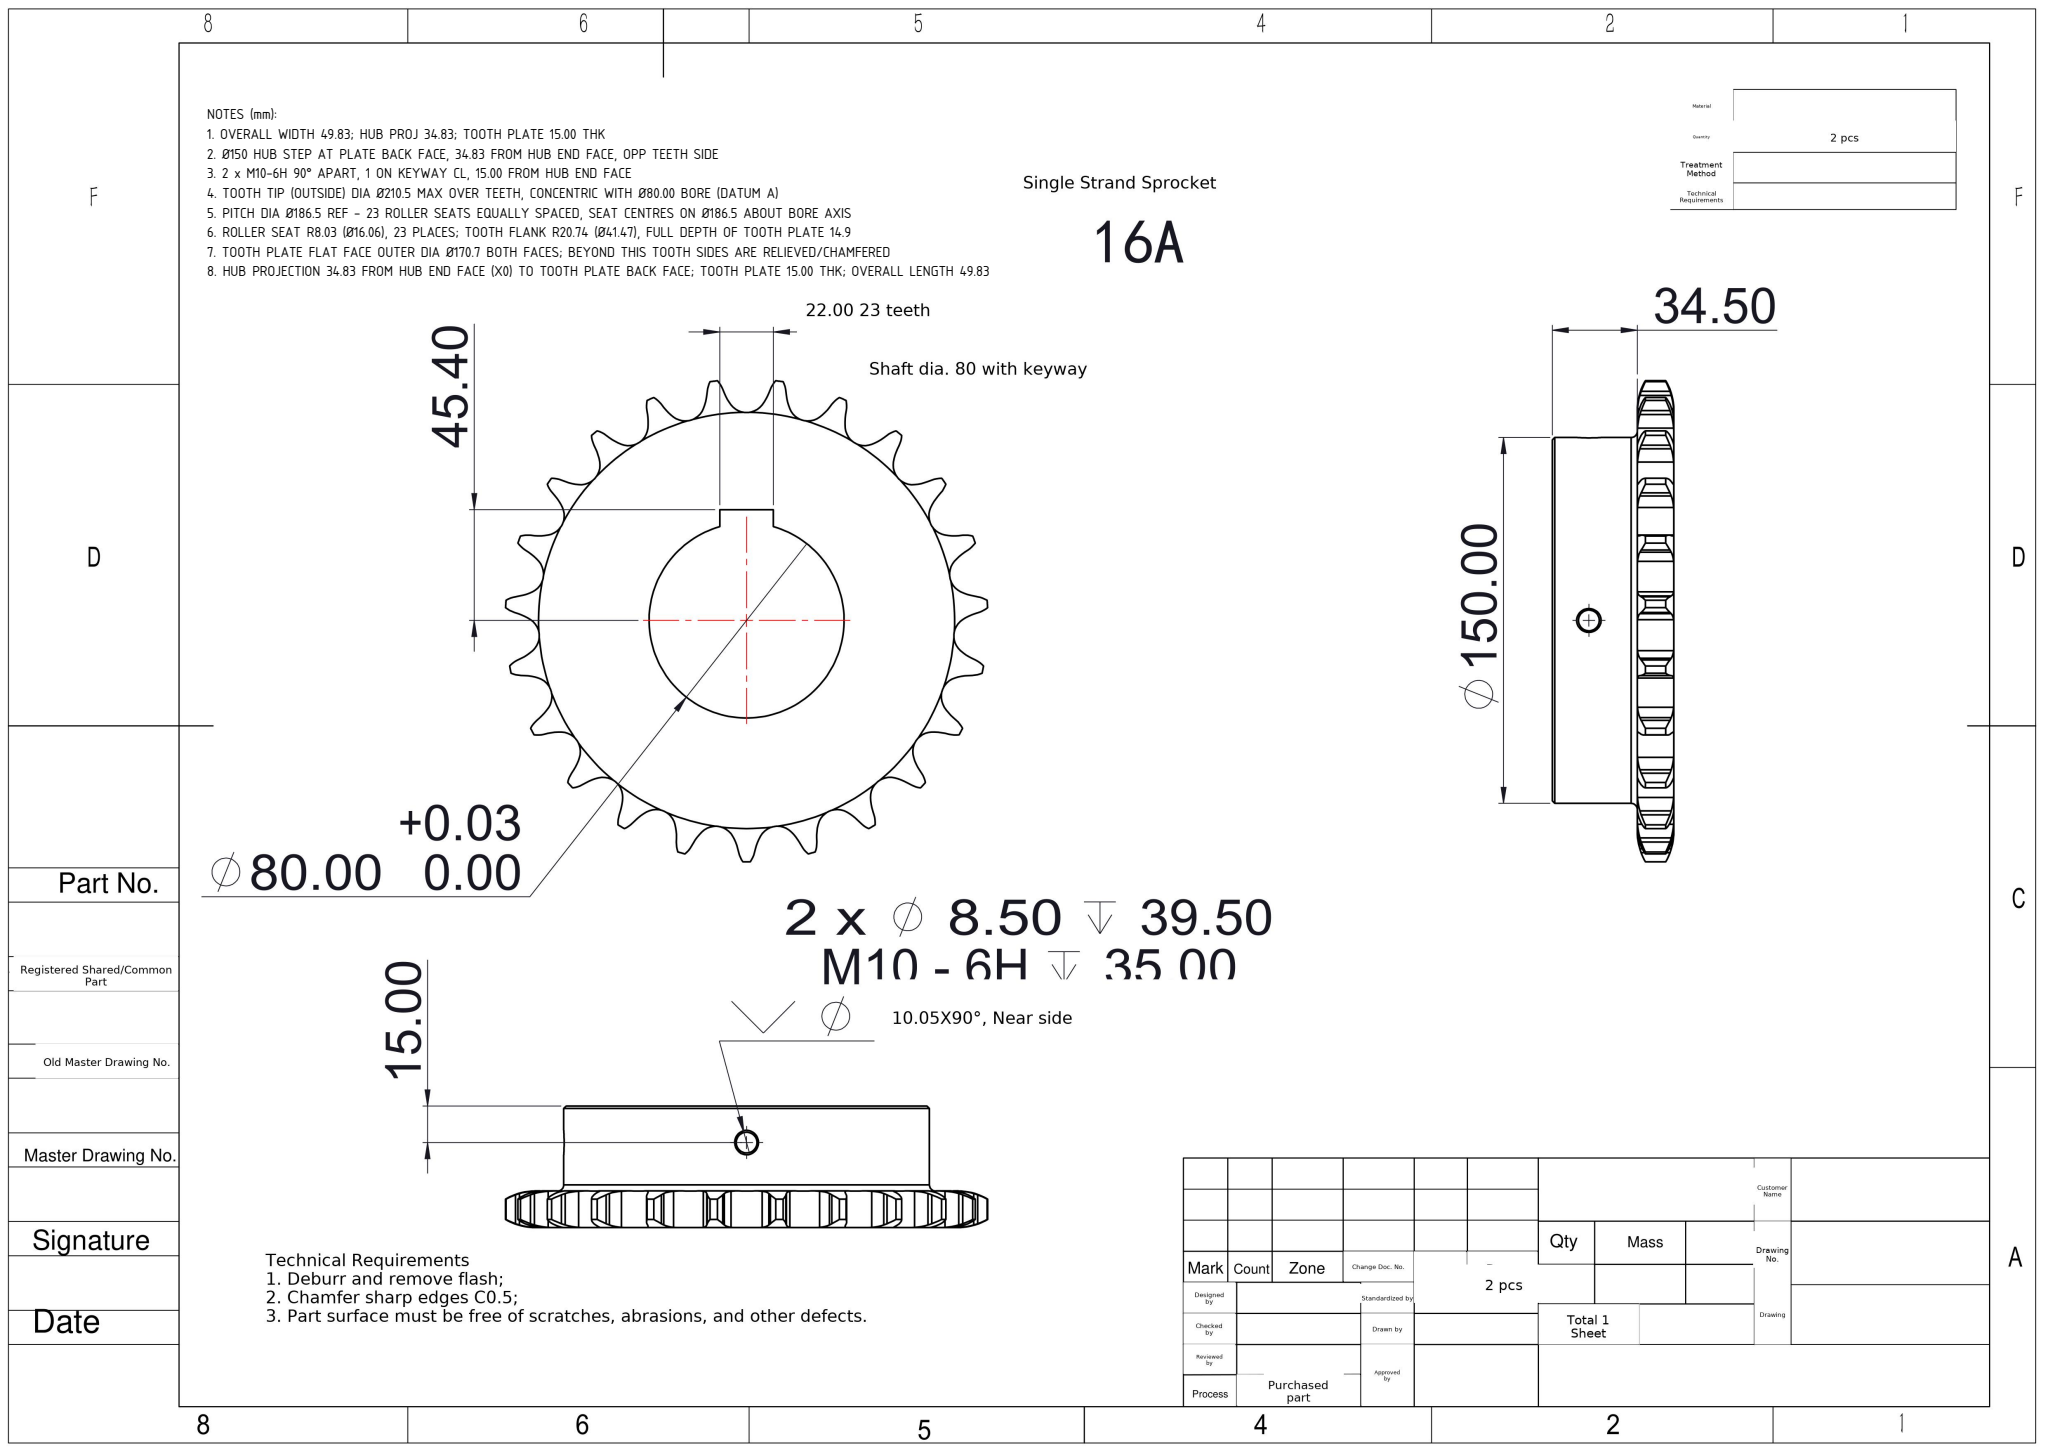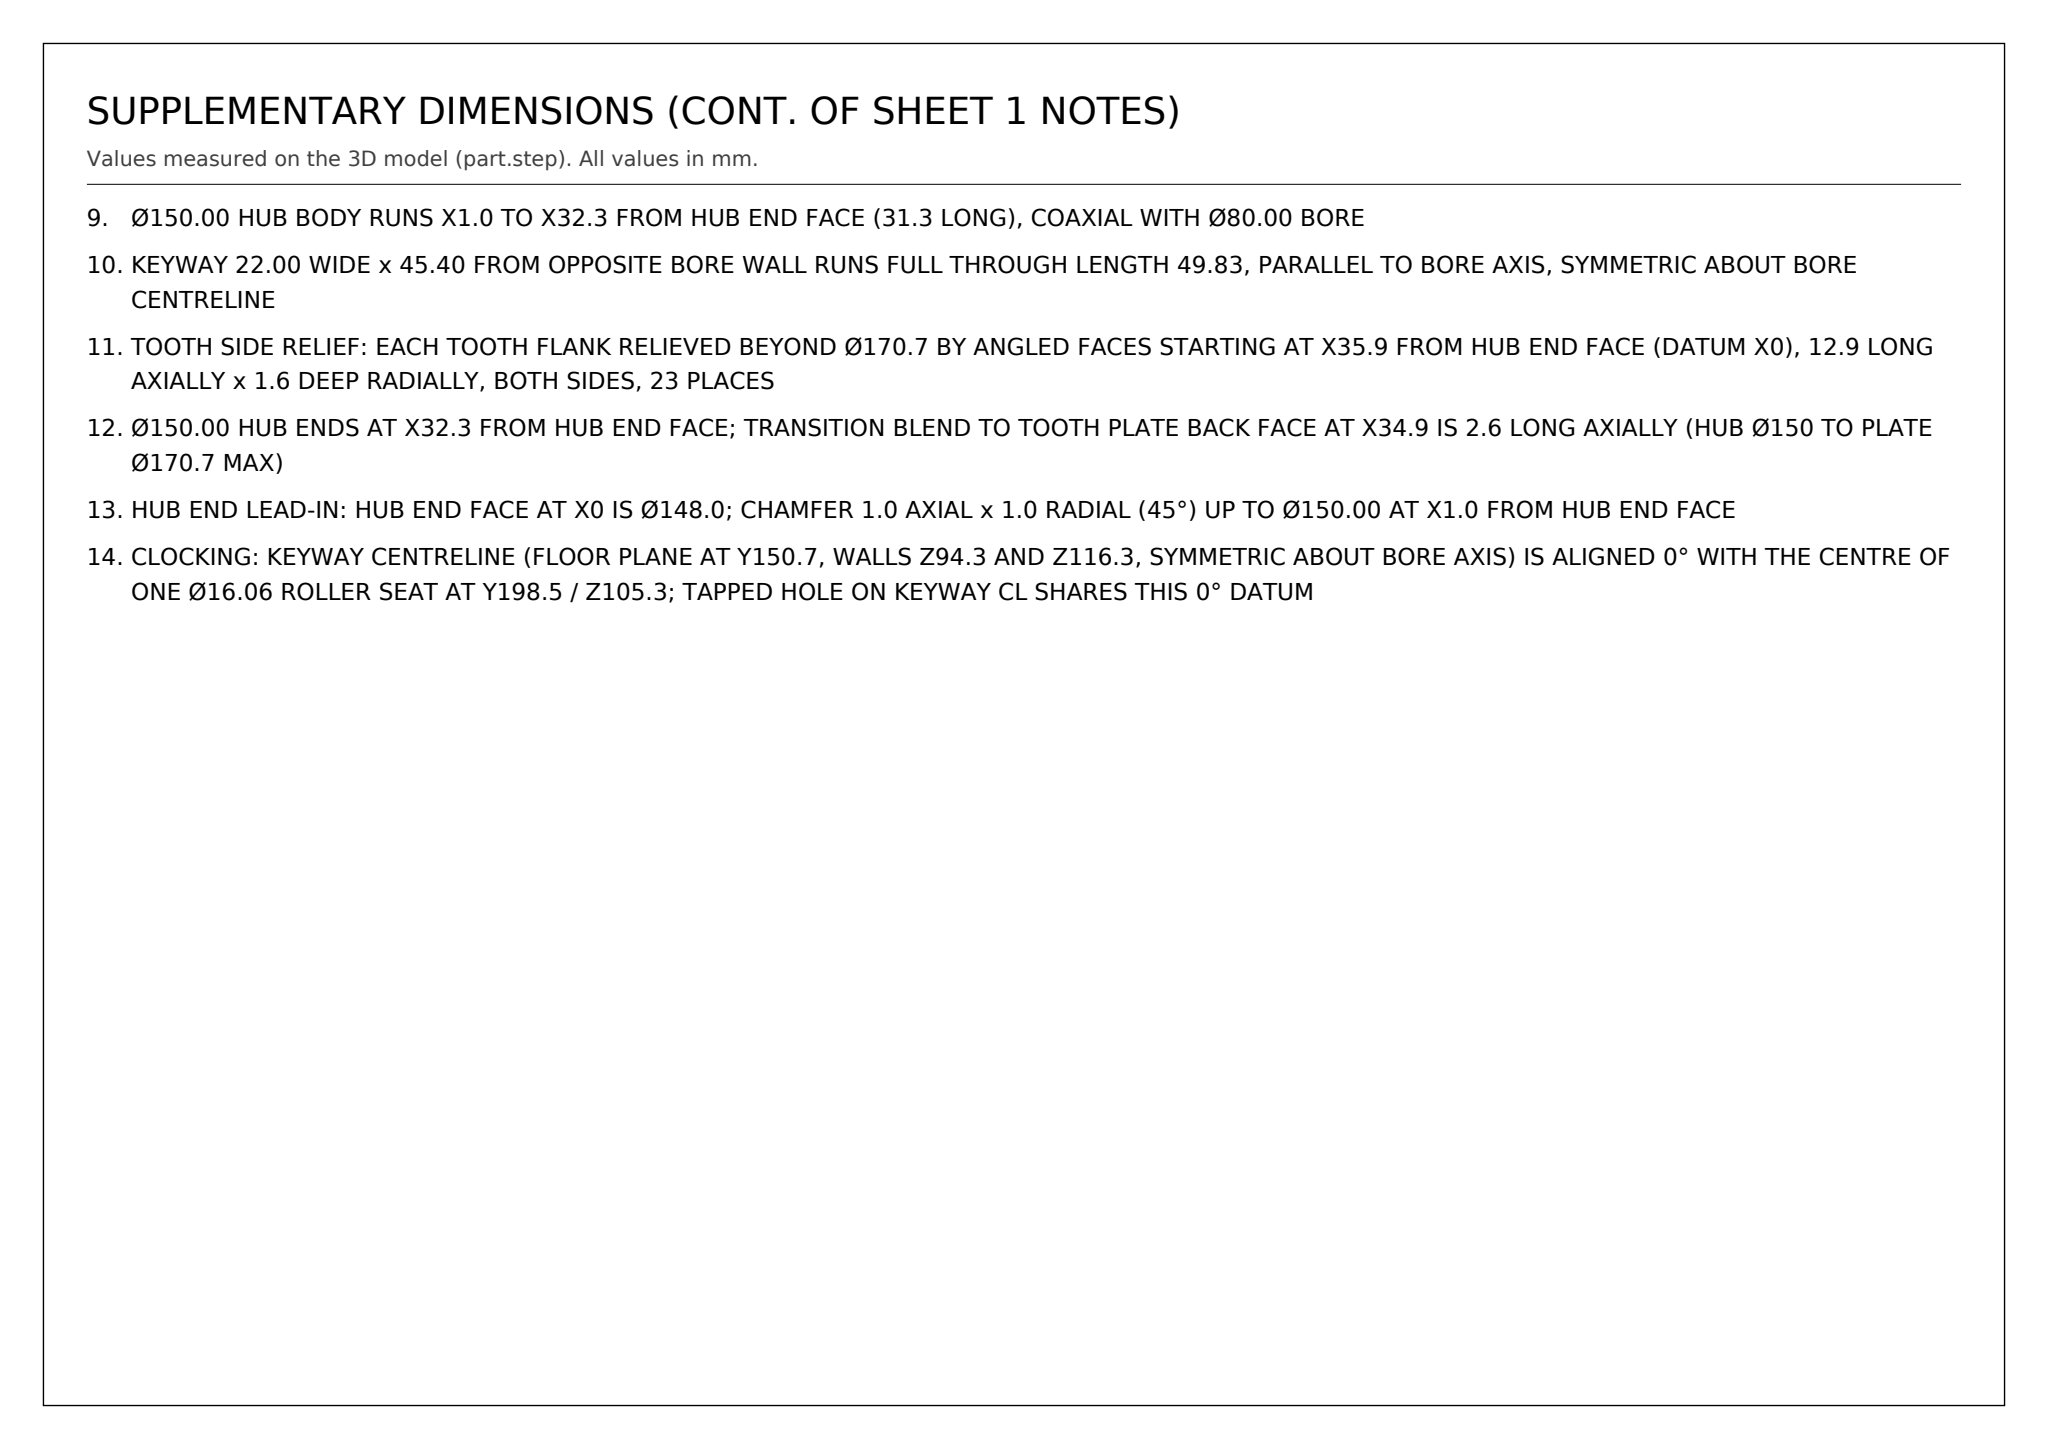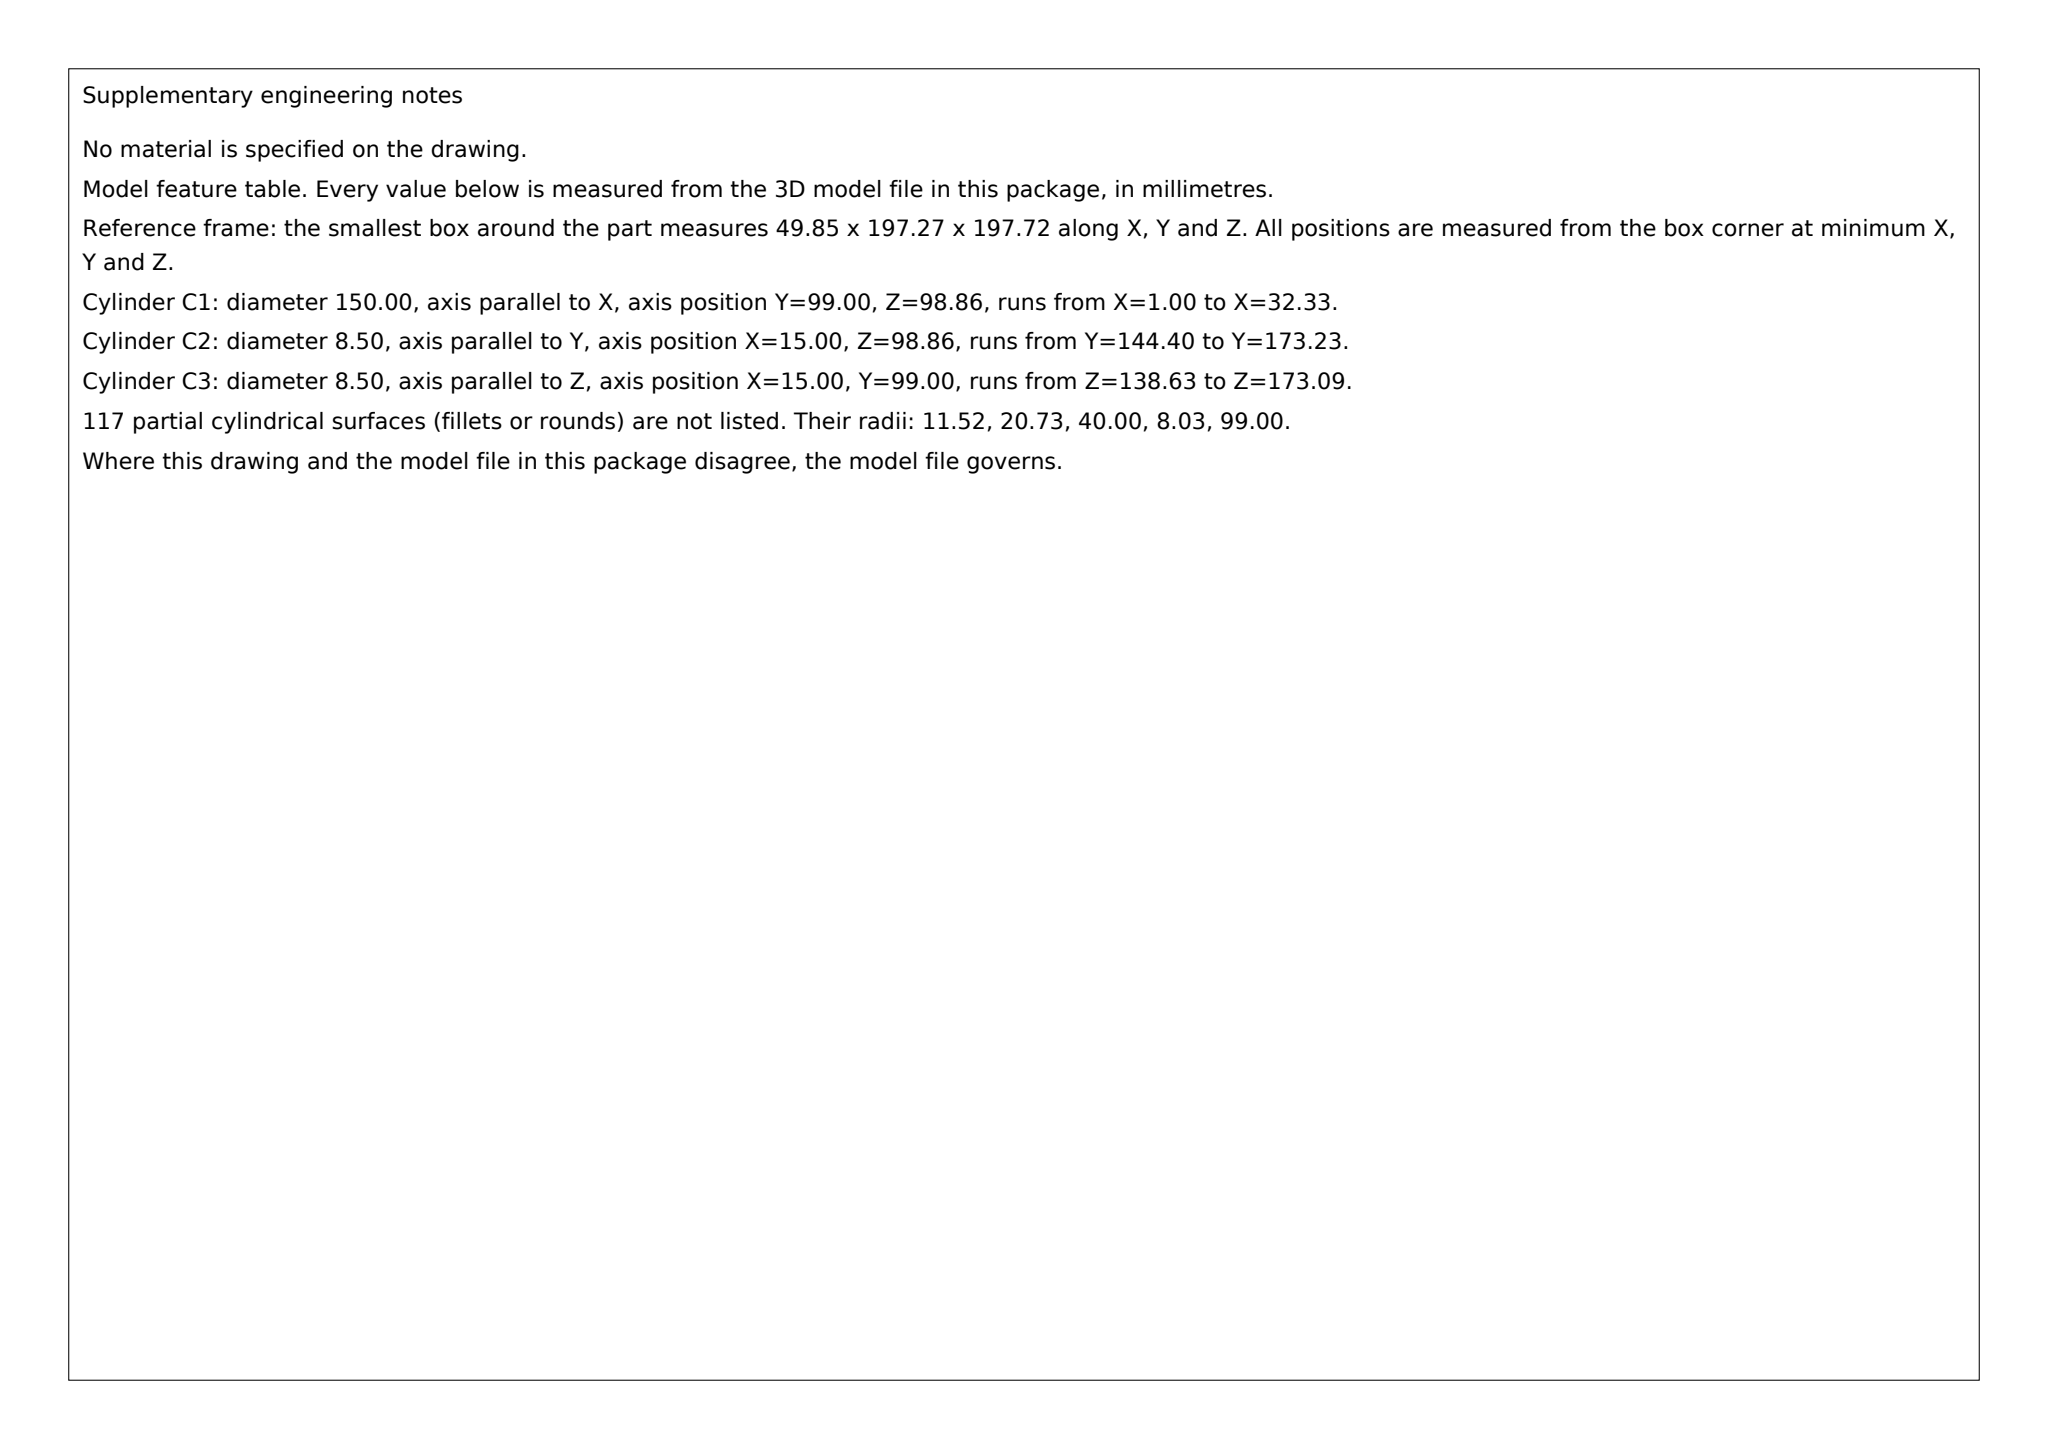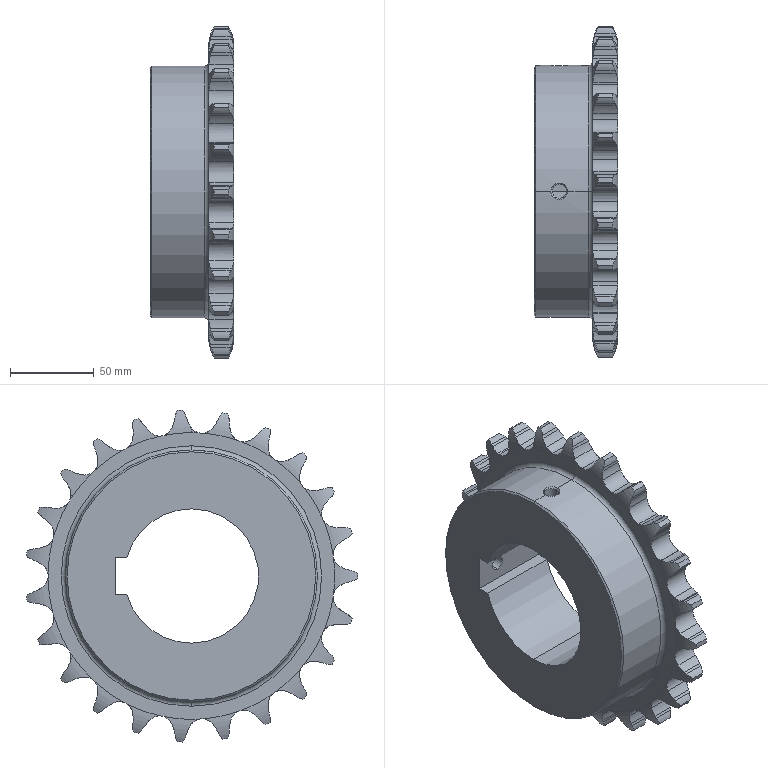Part | SolidWorks | mm | 1 solid | 267 faces | box 49.85 x 197.27 x 197.72 mm | volume 737207 mm3 | cylinder 159 | plane 52 | torus 50 | cone 6 | commonest cylinder face diameters 23.032 x49 41.467 x48 16.059 x30 198 x23 8.5 x4 80 x3 150 x2
Drawing notes:
OVERALL WIDTH 49.83; HUB PROJ 34.83; TOOTH PLATE 15.00 THK | from the solid: x planes 0 / 34.86 / 49.83; bbox x=49.851; tooth-flank cyls Ø16.059 length 15.01
Ø150 HUB STEP AT PLATE BACK FACE, 34.83 FROM HUB END FACE, OPP TEETH SIDE | from the solid: annular face plane x=34.86 between hub (x=0-34.86) and 15.0 thk toothed plate (x=34.86-49.83)
2 x M10-6H 90° APART, 1 ON KEYWAY CL, 15.00 FROM HUB END FACE | from the solid: Ø8.5 holes: axis Y at x=15.0,z=105.27 (keyway CL z=105.27) and axis Z at x=15.0,y=105.27; hub end plane x=0
TOOTH TIP (OUTSIDE) DIA Ø210.5 MAX OVER TEETH, CONCENTRIC WITH Ø80.00 BORE (DATUM A) | from the solid: bbox_xyz y/z = 210.522 / 210.214 (overall across teeth, bore axis at y=105.3, z=105.3)
PITCH DIA Ø186.5 REF - 23 ROLLER SEATS EQUALLY SPACED, SEAT CENTRES ON Ø186.5 ABOUT BORE AXIS | from the solid: roller-seat arcs Ø16.06 centres e.g. (y12.9, z118.0) at radius 93.27 from bore axis (105.3,105.3) => 186.5 dia
ROLLER SEAT R8.03 (Ø16.06), 23 PLACES; TOOTH FLANK R20.74 (Ø41.47), FULL DEPTH OF TOOTH PLATE 14.9 | from the solid: cylinders Ø16.06 and Ø41.47, axis x, from x=34.8/34.9 to x=49.8/49.9
TOOTH PLATE FLAT FACE OUTER DIA Ø170.7 BOTH FACES; BEYOND THIS TOOTH SIDES ARE RELIEVED/CHAMFERED | from the solid: axis_planes x=34.9 and x=49.8, extent y/z [19.9, 190.6] = 170.7 dia; inclined_planes at tooth sides, size 12.9 x 0.3 x 1.6
HUB PROJECTION 34.83 FROM HUB END FACE (X0) TO TOOTH PLATE BACK FACE; TOOTH PLATE 15.00 THK; OVERALL LENGTH 49.83 | from the solid: axis_planes x=0.0 (hub end face), x=34.9 (plate back face), x=49.8 (plate front face); bbox_xyz x = 49.851
Ø150.00 HUB BODY RUNS X1.0 TO X32.3 FROM HUB END FACE (31.3 LONG), COAXIAL WITH Ø80.00 BORE | from the solid: cylinder boss/shaft Ø150.0, axis x, centre (105.3,105.3), from 1.0 to 32.3, 360 deg
KEYWAY 22.00 WIDE x 45.40 FROM OPPOSITE BORE WALL RUNS FULL THROUGH LENGTH 49.83, PARALLEL TO BORE AXIS, SYMMETRIC ABOUT BORE CENTRELINE | from the solid: axis_plane y=150.7 extent x[0.0,49.8], z[94.3,116.3] (22.0 wide, full length); side planes z=116.3 and z=94.3, extent x[0.0,49.8]
TOOTH SIDE RELIEF: EACH TOOTH FLANK RELIEVED BEYOND Ø170.7 BY ANGLED FACES STARTING AT X35.9 FROM HUB END FACE (DATUM X0), 12.9 LONG AXIALLY x 1.6 DEEP RADIALLY, BOTH SIDES, 23 PLACES | from the solid: inclined_planes (tooth side faces) bbox_from [35.9, y, z] size [12.9, 0.3-0.4, 1.6], angles 10.3deg/13.2deg to axes
Ø150.00 HUB ENDS AT X32.3 FROM HUB END FACE; TRANSITION BLEND TO TOOTH PLATE BACK FACE AT X34.9 IS 2.6 LONG AXIALLY (HUB Ø150 TO PLATE Ø170.7 MAX) | from the solid: cylinder boss dia 150.0 axis x from 1.0 to 32.3; axis_plane normal x at offset 34.9 (tooth plate back face)
HUB END LEAD-IN: HUB END FACE AT X0 IS Ø148.0; CHAMFER 1.0 AXIAL x 1.0 RADIAL (45°) UP TO Ø150.00 AT X1.0 FROM HUB END FACE | from the solid: axis_plane normal x offset 0.0 extent y/z 31.3-179.3 (Ø148.0); cylinder dia 150.0 starts at x=1.0
CLOCKING: KEYWAY CENTRELINE (FLOOR PLANE AT Y150.7, WALLS Z94.3 AND Z116.3, SYMMETRIC ABOUT BORE AXIS) IS ALIGNED 0° WITH THE CENTRE OF ONE Ø16.06 ROLLER SEAT AT Y198.5 / Z105.3; TAPPED HOLE ON KEYWAY CL SHARES THIS 0° DATUM | from the solid: axis_planes y=150.7 extent z 94.3-116.3 and z=94.3/116.3 (keyway); cylinder Ø16.06 roller seat at [y 198.5, z 105.3] with bore axis at y/z 105.3